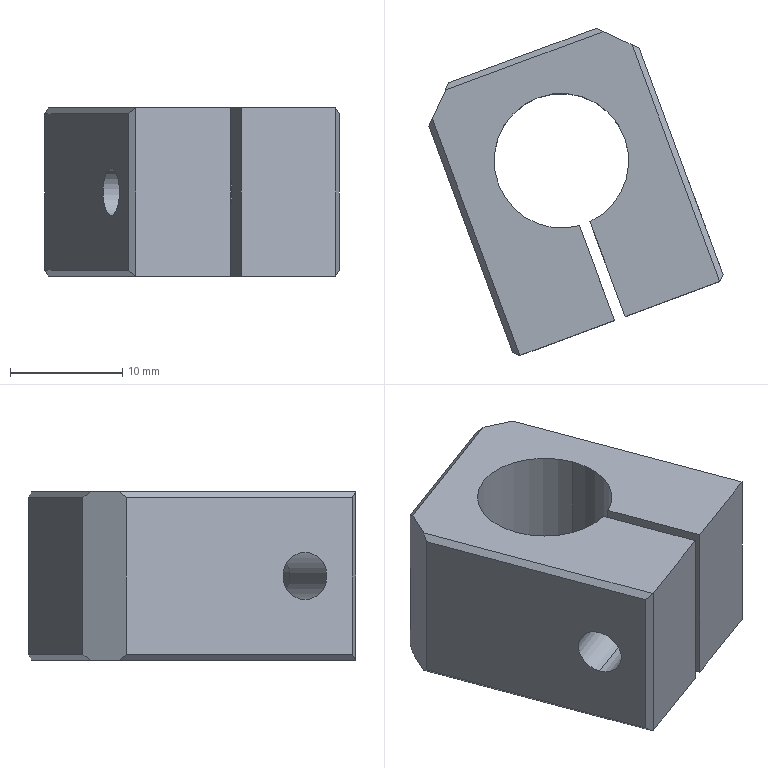Component | SolidWorks | 57-1 | 1 solid | 30 faces | box 26.22 x 29.17 x 15 mm | volume 4970 mm3 | plane 19 | cylinder 9 | cone 2 | commonest cylinder face diameters 12 x3 4.2 x2 8.7 x2 5.3 x2
build123d program:
from build123d import *

# Parameters (mm, degrees)
BOSS_EXTRUDE1_DEPTH   = 15
CHAMFER1_SIZE         = 3
M5_TAPPED_HOLE1_D     = 4.2
M5_TAPPED_HOLE1_DEPTH = 14
M5_TAPPED_HOLE1_TIP   = 1.262
CHAMFER2_SIZE         = 0.5


with BuildPart() as part:
    # Sketch1 → Boss-Extrude1 (new body)
    with BuildSketch(Plane.XY):
        with BuildLine():
            Line((0.5, -5), (10, -5))
            Line((10, -5), (10, 20))
            Line((10, 20), (-10, 20))
            Line((-10, 20), (-10, -5))
            Line((-10, -5), (-0.5, -5))
            Line((-0.5, -5), (-0.5, 4.021))
            ThreePointArc((-0.5, 4.021), (0, 16), (0.5, 4.021))
            Line((0.5, 4.021), (0.5, -5))
        make_face()
    extrude(amount=BOSS_EXTRUDE1_DEPTH)

    # Chamfer1
    chamfer1_edges = [part.edges().sort_by_distance(p)[0] for p in [
        (-10, 20, 7.5),
        (10, 20, 7.5),
    ]]
    chamfer(chamfer1_edges, length=CHAMFER1_SIZE)

    # Sketch2 → Hole1 (revolve, cut)
    with BuildSketch(Plane(origin=(10, 0, 7.5), x_dir=(0, 0, -1), z_dir=(0, 1, 0))):
        Polygon((0, 0), (0, 9.5), (2.65, 9.5), (2.65, 6.021), (4.35, 5), (4.35, 0), align=None)
    revolve(axis=Axis((16.13, 0, 7.5), (-1, 0, 0)), mode=Mode.SUBTRACT)

    # M5 Tapped Hole1
    with Locations(Plane(origin=(-0.5, 0, 0), x_dir=(0, 0, -1), z_dir=(1, 0, 0))):
        with Locations((-7.5, 0)):
            Hole(M5_TAPPED_HOLE1_D / 2, depth=M5_TAPPED_HOLE1_DEPTH)
            with Locations((0, 0, -(M5_TAPPED_HOLE1_DEPTH + M5_TAPPED_HOLE1_TIP / 2))):  # 118° drill point
                Cone(0, M5_TAPPED_HOLE1_D / 2, M5_TAPPED_HOLE1_TIP, mode=Mode.SUBTRACT)

    # Chamfer2
    chamfer2_edges = [part.edges().sort_by_distance(p)[0] for p in [
        (10, -5, 7.5),
        (-10, -5, 7.5),
        (10, 6, 15),
        (-10, 6, 0),
        (-10, 6, 15),
        (0, 20, 0),
        (0, 20, 15),
        (10, 6, 0),
    ]]
    chamfer(chamfer2_edges, length=CHAMFER2_SIZE)


solid = part.part

# Placed as in the assembly
solid = solid.moved(Location((3.473, -47.377, 51.954), (0, 0, 20.325)))
STEP:
#1=COLOUR_RGB('',0.7922,0.8196,0.9333);
#2=FILL_AREA_STYLE_COLOUR('',#1);
#3=FILL_AREA_STYLE('',(#2));
#4=SURFACE_STYLE_FILL_AREA(#3);
#5=SURFACE_SIDE_STYLE('',(#4));
#6=SURFACE_STYLE_USAGE(.BOTH.,#5);
#7=PRESENTATION_STYLE_ASSIGNMENT((#6));
#8=CARTESIAN_POINT('',(-0.2324,-2.002,2.423));
#9=VERTEX_POINT('',#8);
#10=CARTESIAN_POINT('',(-0.2324,-2.002,2.258));
#11=VERTEX_POINT('',#10);
#12=CARTESIAN_POINT('',(-0.2324,-2.002,2.341));
#13=DIRECTION('',(0.9377,0.3473,0.));
#14=DIRECTION('',(-0.3473,0.9377,0.));
#15=AXIS2_PLACEMENT_3D('',#12,#13,#14);
#16=CIRCLE('',#15,0.08268);
#17=EDGE_CURVE('',#9,#11,#16,.T.);
#18=ORIENTED_EDGE('',*,*,#17,.F.);
#19=CARTESIAN_POINT('',(0.1183,-1.872,2.423));
#20=VERTEX_POINT('',#19);
#21=CARTESIAN_POINT('',(0.1183,-1.872,2.423));
#22=DIRECTION('',(0.9377,0.3473,0.));
#23=VECTOR('',#22,39.37);
#24=LINE('',#21,#23);
#25=EDGE_CURVE('',#9,#20,#24,.T.);
#26=ORIENTED_EDGE('',*,*,#25,.T.);
#27=CARTESIAN_POINT('',(0.1183,-1.872,2.258));
#28=VERTEX_POINT('',#27);
#29=CARTESIAN_POINT('',(0.1183,-1.872,2.341));
#30=DIRECTION('',(0.9377,0.3473,0.));
#31=DIRECTION('',(0.,0.,-1.));
#32=AXIS2_PLACEMENT_3D('',#29,#30,#31);
#33=CIRCLE('',#32,0.08268);
#34=EDGE_CURVE('',#20,#28,#33,.T.);
#35=ORIENTED_EDGE('',*,*,#34,.T.);
#36=CARTESIAN_POINT('',(0.1183,-1.872,2.258));
#37=DIRECTION('',(0.9377,0.3473,0.));
#38=VECTOR('',#37,39.37);
#39=LINE('',#36,#38);
#40=EDGE_CURVE('',#11,#28,#39,.T.);
#41=ORIENTED_EDGE('',*,*,#40,.F.);
#42=EDGE_LOOP('',(#18,#26,#35,#41));
#43=FACE_OUTER_BOUND('',#42,.T.);
#44=CARTESIAN_POINT('',(0.1183,-1.872,2.341));
#45=DIRECTION('',(0.9377,0.3473,0.));
#46=DIRECTION('',(0.,0.,-1.));
#47=AXIS2_PLACEMENT_3D('',#44,#45,#46);
#48=CYLINDRICAL_SURFACE('',#47,0.08268);
#49=ADVANCED_FACE('',(#43),#48,.F.);
#50=CARTESIAN_POINT('',(0.3213,-1.797,2.512));
#51=VERTEX_POINT('',#50);
#52=CARTESIAN_POINT('',(0.3213,-1.797,2.169));
#53=VERTEX_POINT('',#52);
#54=CARTESIAN_POINT('',(0.3213,-1.797,2.341));
#55=DIRECTION('',(0.9377,0.3473,0.));
#56=DIRECTION('',(0.,0.,-1.));
#57=AXIS2_PLACEMENT_3D('',#54,#55,#56);
#58=CIRCLE('',#57,0.1713);
#59=EDGE_CURVE('',#51,#53,#58,.T.);
#60=ORIENTED_EDGE('',*,*,#59,.F.);
#61=CARTESIAN_POINT('',(0.5059,-1.728,2.512));
#62=VERTEX_POINT('',#61);
#63=CARTESIAN_POINT('',(0.5059,-1.728,2.512));
#64=DIRECTION('',(0.9377,0.3473,0.));
#65=VECTOR('',#64,39.37);
#66=LINE('',#63,#65);
#67=EDGE_CURVE('',#51,#62,#66,.T.);
#68=ORIENTED_EDGE('',*,*,#67,.T.);
#69=CARTESIAN_POINT('',(0.5059,-1.728,2.169));
#70=VERTEX_POINT('',#69);
#71=CARTESIAN_POINT('',(0.5059,-1.728,2.341));
#72=DIRECTION('',(0.9377,0.3473,0.));
#73=DIRECTION('',(0.,0.,-1.));
#74=AXIS2_PLACEMENT_3D('',#71,#72,#73);
#75=CIRCLE('',#74,0.1713);
#76=EDGE_CURVE('',#62,#70,#75,.T.);
#77=ORIENTED_EDGE('',*,*,#76,.T.);
#78=CARTESIAN_POINT('',(0.5059,-1.728,2.169));
#79=DIRECTION('',(0.9377,0.3473,0.));
#80=VECTOR('',#79,39.37);
#81=LINE('',#78,#80);
#82=EDGE_CURVE('',#53,#70,#81,.T.);
#83=ORIENTED_EDGE('',*,*,#82,.F.);
#84=EDGE_LOOP('',(#60,#68,#77,#83));
#85=FACE_OUTER_BOUND('',#84,.T.);
#86=CARTESIAN_POINT('',(0.5059,-1.728,2.341));
#87=DIRECTION('',(0.9377,0.3473,0.));
#88=DIRECTION('',(0.,0.,-1.));
#89=AXIS2_PLACEMENT_3D('',#86,#87,#88);
#90=CYLINDRICAL_SURFACE('',#89,0.1713);
#91=ADVANCED_FACE('',(#85),#90,.F.);
#92=CARTESIAN_POINT('',(0.2836,-1.811,2.445));
#93=VERTEX_POINT('',#92);
#94=CARTESIAN_POINT('',(0.2836,-1.811,2.236));
#95=VERTEX_POINT('',#94);
#96=CARTESIAN_POINT('',(0.2836,-1.811,2.341));
#97=DIRECTION('',(0.9377,0.3473,0.));
#98=DIRECTION('',(0.,0.,-1.));
#99=AXIS2_PLACEMENT_3D('',#96,#97,#98);
#100=CIRCLE('',#99,0.1043);
#101=EDGE_CURVE('',#93,#95,#100,.T.);
#102=ORIENTED_EDGE('',*,*,#101,.F.);
#103=CARTESIAN_POINT('',(0.3213,-1.797,2.512));
#104=DIRECTION('',(0.483,0.1789,0.8572));
#105=VECTOR('',#104,39.37);
#106=LINE('',#103,#105);
#107=EDGE_CURVE('',#93,#51,#106,.T.);
#108=ORIENTED_EDGE('',*,*,#107,.T.);
#109=ORIENTED_EDGE('',*,*,#59,.T.);
#110=CARTESIAN_POINT('',(0.3213,-1.797,2.169));
#111=DIRECTION('',(0.483,0.1789,-0.8572));
#112=VECTOR('',#111,39.37);
#113=LINE('',#110,#112);
#114=EDGE_CURVE('',#95,#53,#113,.T.);
#115=ORIENTED_EDGE('',*,*,#114,.F.);
#116=EDGE_LOOP('',(#102,#108,#109,#115));
#117=FACE_OUTER_BOUND('',#116,.T.);
#118=CARTESIAN_POINT('',(0.3213,-1.797,2.341));
#119=DIRECTION('',(0.9377,0.3473,0.));
#120=DIRECTION('',(0.,0.,-1.));
#121=AXIS2_PLACEMENT_3D('',#118,#119,#120);
#122=CONICAL_SURFACE('',#121,0.1713,1.03);
#123=ADVANCED_FACE('',(#117),#122,.F.);
#124=CARTESIAN_POINT('',(0.1552,-1.858,2.445));
#125=VERTEX_POINT('',#124);
#126=CARTESIAN_POINT('',(0.1552,-1.858,2.236));
#127=VERTEX_POINT('',#126);
#128=CARTESIAN_POINT('',(0.1552,-1.858,2.341));
#129=DIRECTION('',(0.9377,0.3473,0.));
#130=DIRECTION('',(-0.3473,0.9377,0.));
#131=AXIS2_PLACEMENT_3D('',#128,#129,#130);
#132=CIRCLE('',#131,0.1043);
#133=EDGE_CURVE('',#125,#127,#132,.T.);
#134=ORIENTED_EDGE('',*,*,#133,.F.);
#135=CARTESIAN_POINT('',(0.5059,-1.728,2.445));
#136=DIRECTION('',(0.9377,0.3473,0.));
#137=VECTOR('',#136,39.37);
#138=LINE('',#135,#137);
#139=EDGE_CURVE('',#125,#93,#138,.T.);
#140=ORIENTED_EDGE('',*,*,#139,.T.);
#141=ORIENTED_EDGE('',*,*,#101,.T.);
#142=CARTESIAN_POINT('',(0.5059,-1.728,2.236));
#143=DIRECTION('',(0.9377,0.3473,0.));
#144=VECTOR('',#143,39.37);
#145=LINE('',#142,#144);
#146=EDGE_CURVE('',#127,#95,#145,.T.);
#147=ORIENTED_EDGE('',*,*,#146,.F.);
#148=EDGE_LOOP('',(#134,#140,#141,#147));
#149=FACE_OUTER_BOUND('',#148,.T.);
#150=CARTESIAN_POINT('',(0.5059,-1.728,2.341));
#151=DIRECTION('',(0.9377,0.3473,0.));
#152=DIRECTION('',(0.,0.,-1.));
#153=AXIS2_PLACEMENT_3D('',#150,#151,#152);
#154=CYLINDRICAL_SURFACE('',#153,0.1043);
#155=ADVANCED_FACE('',(#149),#154,.F.);
#156=CARTESIAN_POINT('',(0.2215,-1.414,2.636));
#157=VERTEX_POINT('',#156);
#158=CARTESIAN_POINT('',(0.1002,-1.71,2.636));
#159=VERTEX_POINT('',#158);
#160=CARTESIAN_POINT('',(0.,-1.496,2.636));
#161=DIRECTION('',(0.,0.,-1.));
#162=DIRECTION('',(0.9377,0.3473,0.));
#163=AXIS2_PLACEMENT_3D('',#160,#161,#162);
#164=CIRCLE('',#163,0.2362);
#165=EDGE_CURVE('',#157,#159,#164,.T.);
#166=ORIENTED_EDGE('',*,*,#165,.F.);
#167=CARTESIAN_POINT('',(0.2215,-1.414,2.045));
#168=VERTEX_POINT('',#167);
#169=CARTESIAN_POINT('',(0.2215,-1.414,2.636));
#170=DIRECTION('',(0.,0.,-1.));
#171=VECTOR('',#170,39.37);
#172=LINE('',#169,#171);
#173=EDGE_CURVE('',#157,#168,#172,.T.);
#174=ORIENTED_EDGE('',*,*,#173,.T.);
#175=CARTESIAN_POINT('',(0.1002,-1.71,2.045));
#176=VERTEX_POINT('',#175);
#177=CARTESIAN_POINT('',(0.,-1.496,2.045));
#178=DIRECTION('',(0.,0.,-1.));
#179=DIRECTION('',(0.9377,0.3473,0.));
#180=AXIS2_PLACEMENT_3D('',#177,#178,#179);
#181=CIRCLE('',#180,0.2362);
#182=EDGE_CURVE('',#168,#176,#181,.T.);
#183=ORIENTED_EDGE('',*,*,#182,.T.);
#184=CARTESIAN_POINT('',(0.1002,-1.71,2.636));
#185=DIRECTION('',(0.,0.,-1.));
#186=VECTOR('',#185,39.37);
#187=LINE('',#184,#186);
#188=EDGE_CURVE('',#159,#176,#187,.T.);
#189=ORIENTED_EDGE('',*,*,#188,.F.);
#190=EDGE_LOOP('',(#166,#174,#183,#189));
#191=FACE_OUTER_BOUND('',#190,.T.);
#192=CARTESIAN_POINT('',(0.,-1.496,2.636));
#193=DIRECTION('',(0.,0.,-1.));
#194=DIRECTION('',(-0.9377,-0.3473,0.));
#195=AXIS2_PLACEMENT_3D('',#192,#193,#194);
#196=CYLINDRICAL_SURFACE('',#195,0.2362);
#197=ADVANCED_FACE('',(#191),#196,.F.);
#198=ORIENTED_EDGE('',*,*,#173,.F.);
#199=CARTESIAN_POINT('',(-0.2215,-1.578,2.636));
#200=VERTEX_POINT('',#199);
#201=CARTESIAN_POINT('',(0.,-1.496,2.636));
#202=DIRECTION('',(0.,0.,-1.));
#203=DIRECTION('',(0.9377,0.3473,0.));
#204=AXIS2_PLACEMENT_3D('',#201,#202,#203);
#205=CIRCLE('',#204,0.2362);
#206=EDGE_CURVE('',#200,#157,#205,.T.);
#207=ORIENTED_EDGE('',*,*,#206,.F.);
#208=CARTESIAN_POINT('',(-0.2215,-1.578,2.045));
#209=VERTEX_POINT('',#208);
#210=CARTESIAN_POINT('',(-0.2215,-1.578,2.636));
#211=DIRECTION('',(0.,0.,-1.));
#212=VECTOR('',#211,39.37);
#213=LINE('',#210,#212);
#214=EDGE_CURVE('',#200,#209,#213,.T.);
#215=ORIENTED_EDGE('',*,*,#214,.T.);
#216=CARTESIAN_POINT('',(0.,-1.496,2.045));
#217=DIRECTION('',(0.,0.,-1.));
#218=DIRECTION('',(0.9377,0.3473,0.));
#219=AXIS2_PLACEMENT_3D('',#216,#217,#218);
#220=CIRCLE('',#219,0.2362);
#221=EDGE_CURVE('',#209,#168,#220,.T.);
#222=ORIENTED_EDGE('',*,*,#221,.T.);
#223=EDGE_LOOP('',(#198,#207,#215,#222));
#224=FACE_OUTER_BOUND('',#223,.T.);
#225=CARTESIAN_POINT('',(0.,-1.496,2.636));
#226=DIRECTION('',(0.,0.,-1.));
#227=DIRECTION('',(-0.9377,-0.3473,0.));
#228=AXIS2_PLACEMENT_3D('',#225,#226,#227);
#229=CYLINDRICAL_SURFACE('',#228,0.2362);
#230=ADVANCED_FACE('',(#224),#229,.F.);
#231=CARTESIAN_POINT('',(-0.4649,-1.374,2.616));
#232=VERTEX_POINT('',#231);
#233=CARTESIAN_POINT('',(-0.4649,-1.374,2.065));
#234=VERTEX_POINT('',#233);
#235=CARTESIAN_POINT('',(-0.4649,-1.374,2.636));
#236=DIRECTION('',(0.,0.,-1.));
#237=VECTOR('',#236,39.37);
#238=LINE('',#235,#237);
#239=EDGE_CURVE('',#232,#234,#238,.T.);
#240=ORIENTED_EDGE('',*,*,#239,.T.);
#241=CARTESIAN_POINT('',(-0.1709,-2.168,2.065));
#242=VERTEX_POINT('',#241);
#243=CARTESIAN_POINT('',(-0.5059,-1.264,2.065));
#244=DIRECTION('',(0.3473,-0.9377,0.));
#245=VECTOR('',#244,39.37);
#246=LINE('',#243,#245);
#247=EDGE_CURVE('',#234,#242,#246,.T.);
#248=ORIENTED_EDGE('',*,*,#247,.T.);
#249=CARTESIAN_POINT('',(-0.1709,-2.168,2.616));
#250=VERTEX_POINT('',#249);
#251=CARTESIAN_POINT('',(-0.1709,-2.168,2.636));
#252=DIRECTION('',(0.,0.,1.));
#253=VECTOR('',#252,39.37);
#254=LINE('',#251,#253);
#255=EDGE_CURVE('',#242,#250,#254,.T.);
#256=ORIENTED_EDGE('',*,*,#255,.T.);
#257=CARTESIAN_POINT('',(-0.4649,-1.374,2.616));
#258=DIRECTION('',(-0.3473,0.9377,0.));
#259=VECTOR('',#258,39.37);
#260=LINE('',#257,#259);
#261=EDGE_CURVE('',#250,#232,#260,.T.);
#262=ORIENTED_EDGE('',*,*,#261,.T.);
#263=EDGE_LOOP('',(#240,#248,#256,#262));
#264=FACE_OUTER_BOUND('',#263,.T.);
#265=CARTESIAN_POINT('',(-0.2324,-2.002,2.341));
#266=DIRECTION('',(0.9377,0.3473,0.));
#267=DIRECTION('',(-0.3473,0.9377,0.));
#268=AXIS2_PLACEMENT_3D('',#265,#266,#267);
#269=CIRCLE('',#268,0.08268);
#270=EDGE_CURVE('',#11,#9,#269,.T.);
#271=ORIENTED_EDGE('',*,*,#270,.T.);
#272=ORIENTED_EDGE('',*,*,#17,.T.);
#273=EDGE_LOOP('',(#271,#272));
#274=FACE_BOUND('',#273,.T.);
#275=CARTESIAN_POINT('',(-0.5059,-1.264,2.636));
#276=DIRECTION('',(0.9377,0.3473,0.));
#277=DIRECTION('',(-0.3473,0.9377,0.));
#278=AXIS2_PLACEMENT_3D('',#275,#276,#277);
#279=PLANE('',#278);
#280=ADVANCED_FACE('',(#264,#274),#279,.F.);
#281=CARTESIAN_POINT('',(-0.1456,-2.18,2.636));
#282=VERTEX_POINT('',#281);
#283=CARTESIAN_POINT('',(0.1867,-2.057,2.636));
#284=VERTEX_POINT('',#283);
#285=CARTESIAN_POINT('',(-0.1641,-2.187,2.636));
#286=DIRECTION('',(0.9377,0.3473,0.));
#287=VECTOR('',#286,39.37);
#288=LINE('',#285,#287);
#289=EDGE_CURVE('',#282,#284,#288,.T.);
#290=ORIENTED_EDGE('',*,*,#289,.F.);
#291=CARTESIAN_POINT('',(-0.1456,-2.18,2.045));
#292=VERTEX_POINT('',#291);
#293=CARTESIAN_POINT('',(-0.1456,-2.18,2.636));
#294=DIRECTION('',(0.,0.,-1.));
#295=VECTOR('',#294,39.37);
#296=LINE('',#293,#295);
#297=EDGE_CURVE('',#282,#292,#296,.T.);
#298=ORIENTED_EDGE('',*,*,#297,.T.);
#299=CARTESIAN_POINT('',(0.1867,-2.057,2.045));
#300=VERTEX_POINT('',#299);
#301=CARTESIAN_POINT('',(-0.1641,-2.187,2.045));
#302=DIRECTION('',(0.9377,0.3473,0.));
#303=VECTOR('',#302,39.37);
#304=LINE('',#301,#303);
#305=EDGE_CURVE('',#292,#300,#304,.T.);
#306=ORIENTED_EDGE('',*,*,#305,.T.);
#307=CARTESIAN_POINT('',(0.1867,-2.057,2.636));
#308=DIRECTION('',(0.,0.,-1.));
#309=VECTOR('',#308,39.37);
#310=LINE('',#307,#309);
#311=EDGE_CURVE('',#284,#300,#310,.T.);
#312=ORIENTED_EDGE('',*,*,#311,.F.);
#313=EDGE_LOOP('',(#290,#298,#306,#312));
#314=FACE_OUTER_BOUND('',#313,.T.);
#315=CARTESIAN_POINT('',(-0.1641,-2.187,2.636));
#316=DIRECTION('',(-0.3473,0.9377,0.));
#317=DIRECTION('',(0.,0.,1.));
#318=AXIS2_PLACEMENT_3D('',#315,#316,#317);
#319=PLANE('',#318);
#320=ADVANCED_FACE('',(#314),#319,.F.);
#321=CARTESIAN_POINT('',(0.1183,-1.872,2.341));
#322=DIRECTION('',(0.9377,0.3473,0.));
#323=DIRECTION('',(0.,0.,-1.));
#324=AXIS2_PLACEMENT_3D('',#321,#322,#323);
#325=CIRCLE('',#324,0.08268);
#326=EDGE_CURVE('',#28,#20,#325,.T.);
#327=ORIENTED_EDGE('',*,*,#326,.F.);
#328=ORIENTED_EDGE('',*,*,#34,.F.);
#329=EDGE_LOOP('',(#327,#328));
#330=FACE_BOUND('',#329,.T.);
#331=CARTESIAN_POINT('',(0.06331,-1.724,2.045));
#332=VERTEX_POINT('',#331);
#333=CARTESIAN_POINT('',(0.06331,-1.724,2.045));
#334=DIRECTION('',(-0.3473,0.9377,0.));
#335=VECTOR('',#334,39.37);
#336=LINE('',#333,#335);
#337=EDGE_CURVE('',#300,#332,#336,.T.);
#338=ORIENTED_EDGE('',*,*,#337,.T.);
#339=CARTESIAN_POINT('',(0.06331,-1.724,2.636));
#340=VERTEX_POINT('',#339);
#341=CARTESIAN_POINT('',(0.06331,-1.724,2.636));
#342=DIRECTION('',(0.,0.,-1.));
#343=VECTOR('',#342,39.37);
#344=LINE('',#341,#343);
#345=EDGE_CURVE('',#340,#332,#344,.T.);
#346=ORIENTED_EDGE('',*,*,#345,.F.);
#347=CARTESIAN_POINT('',(0.06331,-1.724,2.636));
#348=DIRECTION('',(-0.3473,0.9377,0.));
#349=VECTOR('',#348,39.37);
#350=LINE('',#347,#349);
#351=EDGE_CURVE('',#284,#340,#350,.T.);
#352=ORIENTED_EDGE('',*,*,#351,.F.);
#353=ORIENTED_EDGE('',*,*,#311,.T.);
#354=EDGE_LOOP('',(#338,#346,#352,#353));
#355=FACE_OUTER_BOUND('',#354,.T.);
#356=CARTESIAN_POINT('',(0.06331,-1.724,2.636));
#357=DIRECTION('',(-0.9377,-0.3473,0.));
#358=DIRECTION('',(0.3473,-0.9377,0.));
#359=AXIS2_PLACEMENT_3D('',#356,#357,#358);
#360=PLANE('',#359);
#361=ADVANCED_FACE('',(#330,#355),#360,.F.);
#362=ORIENTED_EDGE('',*,*,#214,.F.);
#363=CARTESIAN_POINT('',(0.,-1.496,2.636));
#364=DIRECTION('',(0.,0.,-1.));
#365=DIRECTION('',(0.9377,0.3473,0.));
#366=AXIS2_PLACEMENT_3D('',#363,#364,#365);
#367=CIRCLE('',#366,0.2362);
#368=EDGE_CURVE('',#340,#200,#367,.T.);
#369=ORIENTED_EDGE('',*,*,#368,.F.);
#370=ORIENTED_EDGE('',*,*,#345,.T.);
#371=CARTESIAN_POINT('',(0.,-1.496,2.045));
#372=DIRECTION('',(0.,0.,-1.));
#373=DIRECTION('',(0.9377,0.3473,0.));
#374=AXIS2_PLACEMENT_3D('',#371,#372,#373);
#375=CIRCLE('',#374,0.2362);
#376=EDGE_CURVE('',#332,#209,#375,.T.);
#377=ORIENTED_EDGE('',*,*,#376,.T.);
#378=EDGE_LOOP('',(#362,#369,#370,#377));
#379=FACE_OUTER_BOUND('',#378,.T.);
#380=CARTESIAN_POINT('',(0.,-1.496,2.636));
#381=DIRECTION('',(0.,0.,-1.));
#382=DIRECTION('',(-0.9377,-0.3473,0.));
#383=AXIS2_PLACEMENT_3D('',#380,#381,#382);
#384=CYLINDRICAL_SURFACE('',#383,0.2362);
#385=ADVANCED_FACE('',(#379),#384,.F.);
#386=CARTESIAN_POINT('',(0.1552,-1.858,2.341));
#387=DIRECTION('',(0.9377,0.3473,0.));
#388=DIRECTION('',(-0.3473,0.9377,0.));
#389=AXIS2_PLACEMENT_3D('',#386,#387,#388);
#390=CIRCLE('',#389,0.1043);
#391=EDGE_CURVE('',#127,#125,#390,.T.);
#392=ORIENTED_EDGE('',*,*,#391,.T.);
#393=ORIENTED_EDGE('',*,*,#133,.T.);
#394=EDGE_LOOP('',(#392,#393));
#395=FACE_BOUND('',#394,.T.);
#396=CARTESIAN_POINT('',(0.2236,-2.043,2.045));
#397=VERTEX_POINT('',#396);
#398=CARTESIAN_POINT('',(0.1002,-1.71,2.045));
#399=DIRECTION('',(0.3473,-0.9377,0.));
#400=VECTOR('',#399,39.37);
#401=LINE('',#398,#400);
#402=EDGE_CURVE('',#176,#397,#401,.T.);
#403=ORIENTED_EDGE('',*,*,#402,.T.);
#404=CARTESIAN_POINT('',(0.2236,-2.043,2.636));
#405=VERTEX_POINT('',#404);
#406=CARTESIAN_POINT('',(0.2236,-2.043,2.636));
#407=DIRECTION('',(0.,0.,-1.));
#408=VECTOR('',#407,39.37);
#409=LINE('',#406,#408);
#410=EDGE_CURVE('',#405,#397,#409,.T.);
#411=ORIENTED_EDGE('',*,*,#410,.F.);
#412=CARTESIAN_POINT('',(0.1002,-1.71,2.636));
#413=DIRECTION('',(0.3473,-0.9377,0.));
#414=VECTOR('',#413,39.37);
#415=LINE('',#412,#414);
#416=EDGE_CURVE('',#159,#405,#415,.T.);
#417=ORIENTED_EDGE('',*,*,#416,.F.);
#418=ORIENTED_EDGE('',*,*,#188,.T.);
#419=EDGE_LOOP('',(#403,#411,#417,#418));
#420=FACE_OUTER_BOUND('',#419,.T.);
#421=CARTESIAN_POINT('',(0.1002,-1.71,2.636));
#422=DIRECTION('',(0.9377,0.3473,0.));
#423=DIRECTION('',(-0.3473,0.9377,0.));
#424=AXIS2_PLACEMENT_3D('',#421,#422,#423);
#425=PLANE('',#424);
#426=ADVANCED_FACE('',(#395,#420),#425,.F.);
#427=CARTESIAN_POINT('',(0.5559,-1.92,2.045));
#428=VERTEX_POINT('',#427);
#429=CARTESIAN_POINT('',(0.2236,-2.043,2.045));
#430=DIRECTION('',(0.9377,0.3473,0.));
#431=VECTOR('',#430,39.37);
#432=LINE('',#429,#431);
#433=EDGE_CURVE('',#397,#428,#432,.T.);
#434=ORIENTED_EDGE('',*,*,#433,.T.);
#435=CARTESIAN_POINT('',(0.5559,-1.92,2.636));
#436=VERTEX_POINT('',#435);
#437=CARTESIAN_POINT('',(0.5559,-1.92,2.636));
#438=DIRECTION('',(0.,0.,1.));
#439=VECTOR('',#438,39.37);
#440=LINE('',#437,#439);
#441=EDGE_CURVE('',#428,#436,#440,.T.);
#442=ORIENTED_EDGE('',*,*,#441,.T.);
#443=CARTESIAN_POINT('',(0.2236,-2.043,2.636));
#444=DIRECTION('',(0.9377,0.3473,0.));
#445=VECTOR('',#444,39.37);
#446=LINE('',#443,#445);
#447=EDGE_CURVE('',#405,#436,#446,.T.);
#448=ORIENTED_EDGE('',*,*,#447,.F.);
#449=ORIENTED_EDGE('',*,*,#410,.T.);
#450=EDGE_LOOP('',(#434,#442,#448,#449));
#451=FACE_OUTER_BOUND('',#450,.T.);
#452=CARTESIAN_POINT('',(0.2236,-2.043,2.636));
#453=DIRECTION('',(-0.3473,0.9377,0.));
#454=DIRECTION('',(0.,0.,1.));
#455=AXIS2_PLACEMENT_3D('',#452,#453,#454);
#456=PLANE('',#455);
#457=ADVANCED_FACE('',(#451),#456,.F.);
#458=CARTESIAN_POINT('',(0.5059,-1.728,2.341));
#459=DIRECTION('',(0.9377,0.3473,0.));
#460=DIRECTION('',(0.,0.,-1.));
#461=AXIS2_PLACEMENT_3D('',#458,#459,#460);
#462=CIRCLE('',#461,0.1713);
#463=EDGE_CURVE('',#70,#62,#462,.T.);
#464=ORIENTED_EDGE('',*,*,#463,.F.);
#465=ORIENTED_EDGE('',*,*,#76,.F.);
#466=EDGE_LOOP('',(#464,#465));
#467=FACE_BOUND('',#466,.T.);
#468=CARTESIAN_POINT('',(0.5675,-1.895,2.616));
#469=VERTEX_POINT('',#468);
#470=CARTESIAN_POINT('',(0.5675,-1.895,2.065));
#471=VERTEX_POINT('',#470);
#472=CARTESIAN_POINT('',(0.5675,-1.895,2.636));
#473=DIRECTION('',(0.,0.,-1.));
#474=VECTOR('',#473,39.37);
#475=LINE('',#472,#474);
#476=EDGE_CURVE('',#469,#471,#475,.T.);
#477=ORIENTED_EDGE('',*,*,#476,.T.);
#478=CARTESIAN_POINT('',(0.2735,-1.101,2.065));
#479=VERTEX_POINT('',#478);
#480=CARTESIAN_POINT('',(0.2324,-0.9901,2.065));
#481=DIRECTION('',(-0.3473,0.9377,0.));
#482=VECTOR('',#481,39.37);
#483=LINE('',#480,#482);
#484=EDGE_CURVE('',#471,#479,#483,.T.);
#485=ORIENTED_EDGE('',*,*,#484,.T.);
#486=CARTESIAN_POINT('',(0.2735,-1.101,2.616));
#487=VERTEX_POINT('',#486);
#488=CARTESIAN_POINT('',(0.2735,-1.101,2.636));
#489=DIRECTION('',(0.,0.,1.));
#490=VECTOR('',#489,39.37);
#491=LINE('',#488,#490);
#492=EDGE_CURVE('',#479,#487,#491,.T.);
#493=ORIENTED_EDGE('',*,*,#492,.T.);
#494=CARTESIAN_POINT('',(0.5743,-1.913,2.616));
#495=DIRECTION('',(0.3473,-0.9377,0.));
#496=VECTOR('',#495,39.37);
#497=LINE('',#494,#496);
#498=EDGE_CURVE('',#487,#469,#497,.T.);
#499=ORIENTED_EDGE('',*,*,#498,.T.);
#500=EDGE_LOOP('',(#477,#485,#493,#499));
#501=FACE_OUTER_BOUND('',#500,.T.);
#502=CARTESIAN_POINT('',(0.2324,-0.9901,2.636));
#503=DIRECTION('',(-0.9377,-0.3473,0.));
#504=DIRECTION('',(0.3473,-0.9377,0.));
#505=AXIS2_PLACEMENT_3D('',#502,#503,#504);
#506=PLANE('',#505);
#507=ADVANCED_FACE('',(#467,#501),#506,.F.);
#508=CARTESIAN_POINT('',(-0.3952,-1.223,2.065));
#509=VERTEX_POINT('',#508);
#510=CARTESIAN_POINT('',(-0.3952,-1.223,2.616));
#511=VERTEX_POINT('',#510);
#512=CARTESIAN_POINT('',(-0.3952,-1.223,2.636));
#513=DIRECTION('',(0.,0.,1.));
#514=VECTOR('',#513,39.37);
#515=LINE('',#512,#514);
#516=EDGE_CURVE('',#509,#511,#515,.T.);
#517=ORIENTED_EDGE('',*,*,#516,.T.);
#518=CARTESIAN_POINT('',(0.1217,-1.031,2.616));
#519=VERTEX_POINT('',#518);
#520=CARTESIAN_POINT('',(0.1217,-1.031,2.616));
#521=DIRECTION('',(0.9377,0.3473,0.));
#522=VECTOR('',#521,39.37);
#523=LINE('',#520,#522);
#524=EDGE_CURVE('',#511,#519,#523,.T.);
#525=ORIENTED_EDGE('',*,*,#524,.T.);
#526=CARTESIAN_POINT('',(0.1217,-1.031,2.065));
#527=VERTEX_POINT('',#526);
#528=CARTESIAN_POINT('',(0.1217,-1.031,2.636));
#529=DIRECTION('',(0.,0.,-1.));
#530=VECTOR('',#529,39.37);
#531=LINE('',#528,#530);
#532=EDGE_CURVE('',#519,#527,#531,.T.);
#533=ORIENTED_EDGE('',*,*,#532,.T.);
#534=CARTESIAN_POINT('',(-0.5059,-1.264,2.065));
#535=DIRECTION('',(-0.9377,-0.3473,0.));
#536=VECTOR('',#535,39.37);
#537=LINE('',#534,#536);
#538=EDGE_CURVE('',#527,#509,#537,.T.);
#539=ORIENTED_EDGE('',*,*,#538,.T.);
#540=EDGE_LOOP('',(#517,#525,#533,#539));
#541=FACE_OUTER_BOUND('',#540,.T.);
#542=CARTESIAN_POINT('',(-0.5059,-1.264,2.636));
#543=DIRECTION('',(0.3473,-0.9377,0.));
#544=DIRECTION('',(0.,0.,-1.));
#545=AXIS2_PLACEMENT_3D('',#542,#543,#544);
#546=PLANE('',#545);
#547=ADVANCED_FACE('',(#541),#546,.F.);
#548=CARTESIAN_POINT('',(0.2482,-1.089,2.636));
#549=VERTEX_POINT('',#548);
#550=CARTESIAN_POINT('',(0.147,-1.043,2.636));
#551=VERTEX_POINT('',#550);
#552=CARTESIAN_POINT('',(0.1976,-1.066,2.636));
#553=DIRECTION('',(-0.9087,0.4175,0.));
#554=VECTOR('',#553,39.37);
#555=LINE('',#552,#554);
#556=EDGE_CURVE('',#549,#551,#555,.T.);
#557=ORIENTED_EDGE('',*,*,#556,.T.);
#558=CARTESIAN_POINT('',(-0.4068,-1.248,2.636));
#559=VERTEX_POINT('',#558);
#560=CARTESIAN_POINT('',(-0.3883,-1.241,2.636));
#561=DIRECTION('',(-0.9377,-0.3473,0.));
#562=VECTOR('',#561,39.37);
#563=LINE('',#560,#562);
#564=EDGE_CURVE('',#551,#559,#563,.T.);
#565=ORIENTED_EDGE('',*,*,#564,.T.);
#566=CARTESIAN_POINT('',(-0.4533,-1.349,2.636));
#567=VERTEX_POINT('',#566);
#568=CARTESIAN_POINT('',(-0.43,-1.298,2.636));
#569=DIRECTION('',(-0.4175,-0.9087,0.));
#570=VECTOR('',#569,39.37);
#571=LINE('',#568,#570);
#572=EDGE_CURVE('',#559,#567,#571,.T.);
#573=ORIENTED_EDGE('',*,*,#572,.T.);
#574=CARTESIAN_POINT('',(-0.1456,-2.18,2.636));
#575=DIRECTION('',(0.3473,-0.9377,0.));
#576=VECTOR('',#575,39.37);
#577=LINE('',#574,#576);
#578=EDGE_CURVE('',#567,#282,#577,.T.);
#579=ORIENTED_EDGE('',*,*,#578,.T.);
#580=ORIENTED_EDGE('',*,*,#289,.T.);
#581=ORIENTED_EDGE('',*,*,#351,.T.);
#582=ORIENTED_EDGE('',*,*,#368,.T.);
#583=ORIENTED_EDGE('',*,*,#206,.T.);
#584=ORIENTED_EDGE('',*,*,#165,.T.);
#585=ORIENTED_EDGE('',*,*,#416,.T.);
#586=ORIENTED_EDGE('',*,*,#447,.T.);
#587=CARTESIAN_POINT('',(0.255,-1.108,2.636));
#588=DIRECTION('',(-0.3473,0.9377,0.));
#589=VECTOR('',#588,39.37);
#590=LINE('',#587,#589);
#591=EDGE_CURVE('',#436,#549,#590,.T.);
#592=ORIENTED_EDGE('',*,*,#591,.T.);
#593=EDGE_LOOP('',(#557,#565,#573,#579,#580,#581,#582,#583,#584,#585,#586,#592));
#594=FACE_OUTER_BOUND('',#593,.T.);
#595=CARTESIAN_POINT('',(0.,-1.496,2.636));
#596=DIRECTION('',(0.,0.,1.));
#597=DIRECTION('',(0.9377,0.3473,0.));
#598=AXIS2_PLACEMENT_3D('',#595,#596,#597);
#599=PLANE('',#598);
#600=ADVANCED_FACE('',(#594),#599,.T.);
#601=CARTESIAN_POINT('',(-0.4533,-1.349,2.045));
#602=VERTEX_POINT('',#601);
#603=CARTESIAN_POINT('',(-0.4068,-1.248,2.045));
#604=VERTEX_POINT('',#603);
#605=CARTESIAN_POINT('',(-0.4649,-1.374,2.045));
#606=DIRECTION('',(0.4175,0.9087,0.));
#607=VECTOR('',#606,39.37);
#608=LINE('',#605,#607);
#609=EDGE_CURVE('',#602,#604,#608,.T.);
#610=ORIENTED_EDGE('',*,*,#609,.T.);
#611=CARTESIAN_POINT('',(0.147,-1.043,2.045));
#612=VERTEX_POINT('',#611);
#613=CARTESIAN_POINT('',(-0.1299,-1.145,2.045));
#614=DIRECTION('',(0.9377,0.3473,0.));
#615=VECTOR('',#614,39.37);
#616=LINE('',#613,#615);
#617=EDGE_CURVE('',#604,#612,#616,.T.);
#618=ORIENTED_EDGE('',*,*,#617,.T.);
#619=CARTESIAN_POINT('',(0.2482,-1.089,2.045));
#620=VERTEX_POINT('',#619);
#621=CARTESIAN_POINT('',(0.1217,-1.031,2.045));
#622=DIRECTION('',(0.9087,-0.4175,0.));
#623=VECTOR('',#622,39.37);
#624=LINE('',#621,#623);
#625=EDGE_CURVE('',#612,#620,#624,.T.);
#626=ORIENTED_EDGE('',*,*,#625,.T.);
#627=CARTESIAN_POINT('',(0.3507,-1.366,2.045));
#628=DIRECTION('',(0.3473,-0.9377,0.));
#629=VECTOR('',#628,39.37);
#630=LINE('',#627,#629);
#631=EDGE_CURVE('',#620,#428,#630,.T.);
#632=ORIENTED_EDGE('',*,*,#631,.T.);
#633=ORIENTED_EDGE('',*,*,#433,.F.);
#634=ORIENTED_EDGE('',*,*,#402,.F.);
#635=ORIENTED_EDGE('',*,*,#182,.F.);
#636=ORIENTED_EDGE('',*,*,#221,.F.);
#637=ORIENTED_EDGE('',*,*,#376,.F.);
#638=ORIENTED_EDGE('',*,*,#337,.F.);
#639=ORIENTED_EDGE('',*,*,#305,.F.);
#640=CARTESIAN_POINT('',(-0.3507,-1.626,2.045));
#641=DIRECTION('',(-0.3473,0.9377,0.));
#642=VECTOR('',#641,39.37);
#643=LINE('',#640,#642);
#644=EDGE_CURVE('',#292,#602,#643,.T.);
#645=ORIENTED_EDGE('',*,*,#644,.T.);
#646=EDGE_LOOP('',(#610,#618,#626,#632,#633,#634,#635,#636,#637,#638,#639,#645));
#647=FACE_OUTER_BOUND('',#646,.T.);
#648=CARTESIAN_POINT('',(0.,-1.496,2.045));
#649=DIRECTION('',(0.,0.,1.));
#650=DIRECTION('',(0.9377,0.3473,0.));
#651=AXIS2_PLACEMENT_3D('',#648,#649,#650);
#652=PLANE('',#651);
#653=ADVANCED_FACE('',(#647),#652,.F.);
#654=ORIENTED_EDGE('',*,*,#572,.F.);
#655=CARTESIAN_POINT('',(-0.4455,-1.332,2.702));
#656=DIRECTION('',(0.3409,0.7419,-0.5774));
#657=VECTOR('',#656,39.37);
#658=LINE('',#655,#657);
#659=EDGE_CURVE('',#559,#511,#658,.T.);
#660=ORIENTED_EDGE('',*,*,#659,.T.);
#661=ORIENTED_EDGE('',*,*,#516,.F.);
#662=CARTESIAN_POINT('',(-0.3293,-1.079,2.177));
#663=DIRECTION('',(-0.3409,-0.7419,-0.5774));
#664=VECTOR('',#663,39.37);
#665=LINE('',#662,#664);
#666=EDGE_CURVE('',#509,#604,#665,.T.);
#667=ORIENTED_EDGE('',*,*,#666,.T.);
#668=ORIENTED_EDGE('',*,*,#609,.F.);
#669=CARTESIAN_POINT('',(-0.5773,-1.619,2.255));
#670=DIRECTION('',(-0.3409,-0.7419,0.5774));
#671=VECTOR('',#670,39.37);
#672=LINE('',#669,#671);
#673=EDGE_CURVE('',#602,#234,#672,.T.);
#674=ORIENTED_EDGE('',*,*,#673,.T.);
#675=ORIENTED_EDGE('',*,*,#239,.F.);
#676=CARTESIAN_POINT('',(-0.461,-1.366,2.623));
#677=DIRECTION('',(0.3409,0.7419,0.5774));
#678=VECTOR('',#677,39.37);
#679=LINE('',#676,#678);
#680=EDGE_CURVE('',#232,#567,#679,.T.);
#681=ORIENTED_EDGE('',*,*,#680,.T.);
#682=EDGE_LOOP('',(#654,#660,#661,#667,#668,#674,#675,#681));
#683=FACE_OUTER_BOUND('',#682,.T.);
#684=CARTESIAN_POINT('',(-0.4649,-1.374,2.636));
#685=DIRECTION('',(0.9087,-0.4175,0.));
#686=DIRECTION('',(0.,0.,-1.));
#687=AXIS2_PLACEMENT_3D('',#684,#685,#686);
#688=PLANE('',#687);
#689=ADVANCED_FACE('',(#683),#688,.F.);
#690=ORIENTED_EDGE('',*,*,#532,.F.);
#691=CARTESIAN_POINT('',(0.1301,-1.035,2.623));
#692=DIRECTION('',(0.7419,-0.3409,0.5774));
#693=VECTOR('',#692,39.37);
#694=LINE('',#691,#693);
#695=EDGE_CURVE('',#519,#551,#694,.T.);
#696=ORIENTED_EDGE('',*,*,#695,.T.);
#697=ORIENTED_EDGE('',*,*,#556,.F.);
#698=CARTESIAN_POINT('',(0.1638,-1.051,2.702));
#699=DIRECTION('',(0.7419,-0.3409,-0.5774));
#700=VECTOR('',#699,39.37);
#701=LINE('',#698,#700);
#702=EDGE_CURVE('',#549,#487,#701,.T.);
#703=ORIENTED_EDGE('',*,*,#702,.T.);
#704=ORIENTED_EDGE('',*,*,#492,.F.);
#705=CARTESIAN_POINT('',(0.4168,-1.167,2.177));
#706=DIRECTION('',(-0.7419,0.3409,-0.5774));
#707=VECTOR('',#706,39.37);
#708=LINE('',#705,#707);
#709=EDGE_CURVE('',#479,#620,#708,.T.);
#710=ORIENTED_EDGE('',*,*,#709,.T.);
#711=ORIENTED_EDGE('',*,*,#625,.F.);
#712=CARTESIAN_POINT('',(-0.1229,-0.9188,2.255));
#713=DIRECTION('',(-0.7419,0.3409,0.5774));
#714=VECTOR('',#713,39.37);
#715=LINE('',#712,#714);
#716=EDGE_CURVE('',#612,#527,#715,.T.);
#717=ORIENTED_EDGE('',*,*,#716,.T.);
#718=EDGE_LOOP('',(#690,#696,#697,#703,#704,#710,#711,#717));
#719=FACE_OUTER_BOUND('',#718,.T.);
#720=CARTESIAN_POINT('',(0.1217,-1.031,2.636));
#721=DIRECTION('',(-0.4175,-0.9087,0.));
#722=DIRECTION('',(0.,0.,-1.));
#723=AXIS2_PLACEMENT_3D('',#720,#721,#722);
#724=PLANE('',#723);
#725=ADVANCED_FACE('',(#719),#724,.F.);
#726=ORIENTED_EDGE('',*,*,#139,.F.);
#727=ORIENTED_EDGE('',*,*,#391,.F.);
#728=ORIENTED_EDGE('',*,*,#146,.T.);
#729=CARTESIAN_POINT('',(0.2836,-1.811,2.341));
#730=DIRECTION('',(0.9377,0.3473,0.));
#731=DIRECTION('',(0.,0.,-1.));
#732=AXIS2_PLACEMENT_3D('',#729,#730,#731);
#733=CIRCLE('',#732,0.1043);
#734=EDGE_CURVE('',#95,#93,#733,.T.);
#735=ORIENTED_EDGE('',*,*,#734,.T.);
#736=EDGE_LOOP('',(#726,#727,#728,#735));
#737=FACE_OUTER_BOUND('',#736,.T.);
#738=CARTESIAN_POINT('',(0.5059,-1.728,2.341));
#739=DIRECTION('',(0.9377,0.3473,0.));
#740=DIRECTION('',(0.,0.,-1.));
#741=AXIS2_PLACEMENT_3D('',#738,#739,#740);
#742=CYLINDRICAL_SURFACE('',#741,0.1043);
#743=ADVANCED_FACE('',(#737),#742,.F.);
#744=ORIENTED_EDGE('',*,*,#107,.F.);
#745=ORIENTED_EDGE('',*,*,#734,.F.);
#746=ORIENTED_EDGE('',*,*,#114,.T.);
#747=CARTESIAN_POINT('',(0.3213,-1.797,2.341));
#748=DIRECTION('',(0.9377,0.3473,0.));
#749=DIRECTION('',(0.,0.,-1.));
#750=AXIS2_PLACEMENT_3D('',#747,#748,#749);
#751=CIRCLE('',#750,0.1713);
#752=EDGE_CURVE('',#53,#51,#751,.T.);
#753=ORIENTED_EDGE('',*,*,#752,.T.);
#754=EDGE_LOOP('',(#744,#745,#746,#753));
#755=FACE_OUTER_BOUND('',#754,.T.);
#756=CARTESIAN_POINT('',(0.3213,-1.797,2.341));
#757=DIRECTION('',(0.9377,0.3473,0.));
#758=DIRECTION('',(0.,0.,-1.));
#759=AXIS2_PLACEMENT_3D('',#756,#757,#758);
#760=CONICAL_SURFACE('',#759,0.1713,1.03);
#761=ADVANCED_FACE('',(#755),#760,.F.);
#762=ORIENTED_EDGE('',*,*,#67,.F.);
#763=ORIENTED_EDGE('',*,*,#752,.F.);
#764=ORIENTED_EDGE('',*,*,#82,.T.);
#765=ORIENTED_EDGE('',*,*,#463,.T.);
#766=EDGE_LOOP('',(#762,#763,#764,#765));
#767=FACE_OUTER_BOUND('',#766,.T.);
#768=CARTESIAN_POINT('',(0.5059,-1.728,2.341));
#769=DIRECTION('',(0.9377,0.3473,0.));
#770=DIRECTION('',(0.,0.,-1.));
#771=AXIS2_PLACEMENT_3D('',#768,#769,#770);
#772=CYLINDRICAL_SURFACE('',#771,0.1713);
#773=ADVANCED_FACE('',(#767),#772,.F.);
#774=ORIENTED_EDGE('',*,*,#25,.F.);
#775=ORIENTED_EDGE('',*,*,#270,.F.);
#776=ORIENTED_EDGE('',*,*,#40,.T.);
#777=ORIENTED_EDGE('',*,*,#326,.T.);
#778=EDGE_LOOP('',(#774,#775,#776,#777));
#779=FACE_OUTER_BOUND('',#778,.T.);
#780=CARTESIAN_POINT('',(0.1183,-1.872,2.341));
#781=DIRECTION('',(0.9377,0.3473,0.));
#782=DIRECTION('',(0.,0.,-1.));
#783=AXIS2_PLACEMENT_3D('',#780,#781,#782);
#784=CYLINDRICAL_SURFACE('',#783,0.08268);
#785=ADVANCED_FACE('',(#779),#784,.F.);
#786=ORIENTED_EDGE('',*,*,#695,.F.);
#787=ORIENTED_EDGE('',*,*,#524,.F.);
#788=ORIENTED_EDGE('',*,*,#659,.F.);
#789=ORIENTED_EDGE('',*,*,#564,.F.);
#790=EDGE_LOOP('',(#786,#787,#788,#789));
#791=FACE_OUTER_BOUND('',#790,.T.);
#792=CARTESIAN_POINT('',(-0.1299,-1.145,2.636));
#793=DIRECTION('',(-0.2456,0.6631,0.7071));
#794=DIRECTION('',(0.9377,0.3473,0.));
#795=AXIS2_PLACEMENT_3D('',#792,#793,#794);
#796=PLANE('',#795);
#797=ADVANCED_FACE('',(#791),#796,.T.);
#798=ORIENTED_EDGE('',*,*,#716,.F.);
#799=ORIENTED_EDGE('',*,*,#617,.F.);
#800=ORIENTED_EDGE('',*,*,#666,.F.);
#801=ORIENTED_EDGE('',*,*,#538,.F.);
#802=EDGE_LOOP('',(#798,#799,#800,#801));
#803=FACE_OUTER_BOUND('',#802,.T.);
#804=CARTESIAN_POINT('',(-0.5059,-1.264,2.065));
#805=DIRECTION('',(0.2456,-0.6631,0.7071));
#806=DIRECTION('',(-0.9377,-0.3473,0.));
#807=AXIS2_PLACEMENT_3D('',#804,#805,#806);
#808=PLANE('',#807);
#809=ADVANCED_FACE('',(#803),#808,.F.);
#810=ORIENTED_EDGE('',*,*,#680,.F.);
#811=ORIENTED_EDGE('',*,*,#261,.F.);
#812=CARTESIAN_POINT('',(-0.1456,-2.18,2.636));
#813=DIRECTION('',(-0.7419,0.3409,-0.5774));
#814=VECTOR('',#813,39.37);
#815=LINE('',#812,#814);
#816=EDGE_CURVE('',#282,#250,#815,.T.);
#817=ORIENTED_EDGE('',*,*,#816,.F.);
#818=ORIENTED_EDGE('',*,*,#578,.F.);
#819=EDGE_LOOP('',(#810,#811,#817,#818));
#820=FACE_OUTER_BOUND('',#819,.T.);
#821=CARTESIAN_POINT('',(-0.3507,-1.626,2.636));
#822=DIRECTION('',(-0.6631,-0.2456,0.7071));
#823=DIRECTION('',(-0.3473,0.9377,0.));
#824=AXIS2_PLACEMENT_3D('',#821,#822,#823);
#825=PLANE('',#824);
#826=ADVANCED_FACE('',(#820),#825,.T.);
#827=ORIENTED_EDGE('',*,*,#816,.T.);
#828=ORIENTED_EDGE('',*,*,#255,.F.);
#829=CARTESIAN_POINT('',(-0.3986,-2.064,2.242));
#830=DIRECTION('',(-0.7419,0.3409,0.5774));
#831=VECTOR('',#830,39.37);
#832=LINE('',#829,#831);
#833=EDGE_CURVE('',#292,#242,#832,.T.);
#834=ORIENTED_EDGE('',*,*,#833,.F.);
#835=ORIENTED_EDGE('',*,*,#297,.F.);
#836=EDGE_LOOP('',(#827,#828,#834,#835));
#837=FACE_OUTER_BOUND('',#836,.T.);
#838=CARTESIAN_POINT('',(-0.1456,-2.18,2.636));
#839=DIRECTION('',(0.4175,0.9087,0.));
#840=DIRECTION('',(0.,0.,-1.));
#841=AXIS2_PLACEMENT_3D('',#838,#839,#840);
#842=PLANE('',#841);
#843=ADVANCED_FACE('',(#837),#842,.F.);
#844=ORIENTED_EDGE('',*,*,#673,.F.);
#845=ORIENTED_EDGE('',*,*,#644,.F.);
#846=ORIENTED_EDGE('',*,*,#833,.T.);
#847=ORIENTED_EDGE('',*,*,#247,.F.);
#848=EDGE_LOOP('',(#844,#845,#846,#847));
#849=FACE_OUTER_BOUND('',#848,.T.);
#850=CARTESIAN_POINT('',(-0.5059,-1.264,2.065));
#851=DIRECTION('',(0.6631,0.2456,0.7071));
#852=DIRECTION('',(0.3473,-0.9377,0.));
#853=AXIS2_PLACEMENT_3D('',#850,#851,#852);
#854=PLANE('',#853);
#855=ADVANCED_FACE('',(#849),#854,.F.);
#856=ORIENTED_EDGE('',*,*,#702,.F.);
#857=ORIENTED_EDGE('',*,*,#591,.F.);
#858=CARTESIAN_POINT('',(0.6721,-1.667,2.439));
#859=DIRECTION('',(-0.3409,-0.7419,0.5774));
#860=VECTOR('',#859,39.37);
#861=LINE('',#858,#860);
#862=EDGE_CURVE('',#469,#436,#861,.T.);
#863=ORIENTED_EDGE('',*,*,#862,.F.);
#864=ORIENTED_EDGE('',*,*,#498,.F.);
#865=EDGE_LOOP('',(#856,#857,#863,#864));
#866=FACE_OUTER_BOUND('',#865,.T.);
#867=CARTESIAN_POINT('',(0.3507,-1.366,2.636));
#868=DIRECTION('',(0.6631,0.2456,0.7071));
#869=DIRECTION('',(0.3473,-0.9377,0.));
#870=AXIS2_PLACEMENT_3D('',#867,#868,#869);
#871=PLANE('',#870);
#872=ADVANCED_FACE('',(#866),#871,.T.);
#873=ORIENTED_EDGE('',*,*,#862,.T.);
#874=ORIENTED_EDGE('',*,*,#441,.F.);
#875=CARTESIAN_POINT('',(0.6798,-1.65,2.255));
#876=DIRECTION('',(-0.3409,-0.7419,-0.5774));
#877=VECTOR('',#876,39.37);
#878=LINE('',#875,#877);
#879=EDGE_CURVE('',#471,#428,#878,.T.);
#880=ORIENTED_EDGE('',*,*,#879,.F.);
#881=ORIENTED_EDGE('',*,*,#476,.F.);
#882=EDGE_LOOP('',(#873,#874,#880,#881));
#883=FACE_OUTER_BOUND('',#882,.T.);
#884=CARTESIAN_POINT('',(0.5675,-1.895,2.636));
#885=DIRECTION('',(-0.9087,0.4175,0.));
#886=DIRECTION('',(0.,0.,-1.));
#887=AXIS2_PLACEMENT_3D('',#884,#885,#886);
#888=PLANE('',#887);
#889=ADVANCED_FACE('',(#883),#888,.F.);
#890=ORIENTED_EDGE('',*,*,#879,.T.);
#891=ORIENTED_EDGE('',*,*,#631,.F.);
#892=ORIENTED_EDGE('',*,*,#709,.F.);
#893=ORIENTED_EDGE('',*,*,#484,.F.);
#894=EDGE_LOOP('',(#890,#891,#892,#893));
#895=FACE_OUTER_BOUND('',#894,.T.);
#896=CARTESIAN_POINT('',(0.2324,-0.9901,2.065));
#897=DIRECTION('',(-0.6631,-0.2456,0.7071));
#898=DIRECTION('',(-0.3473,0.9377,0.));
#899=AXIS2_PLACEMENT_3D('',#896,#897,#898);
#900=PLANE('',#899);
#901=ADVANCED_FACE('',(#895),#900,.F.);
#902=CLOSED_SHELL('',(#49,#91,#123,#155,#197,#230,#280,#320,#361,#385,#426,#457,#507,#547,#600,#653,#689,#725,#743,#761,#773,#785,#797,#809,#826,#843,#855,#872,#889,#901));
#903=MANIFOLD_SOLID_BREP('',#902);
#904=STYLED_ITEM('',(#7),#903);
#905=(LENGTH_UNIT()NAMED_UNIT(*)SI_UNIT($,.METRE.));
#906=LENGTH_MEASURE_WITH_UNIT(LENGTH_MEASURE(0.0254),#905);
#907=DIMENSIONAL_EXPONENTS(1.,0.,0.,0.,0.,0.,0.);
#908=(CONVERSION_BASED_UNIT('',#906)LENGTH_UNIT()NAMED_UNIT(#907));
#909=UNCERTAINTY_MEASURE_WITH_UNIT(LENGTH_MEASURE(0.00001),#908,'','');
#910=(NAMED_UNIT(*)PLANE_ANGLE_UNIT()SI_UNIT($,.RADIAN.));
#911=(NAMED_UNIT(*)SI_UNIT($,.STERADIAN.)SOLID_ANGLE_UNIT());
#912=(GEOMETRIC_REPRESENTATION_CONTEXT(3)GLOBAL_UNCERTAINTY_ASSIGNED_CONTEXT((#909))GLOBAL_UNIT_ASSIGNED_CONTEXT((#908,#910,#911))REPRESENTATION_CONTEXT('',''));
#913=MECHANICAL_DESIGN_GEOMETRIC_PRESENTATION_REPRESENTATION('',(#904),#912);
#914=CARTESIAN_POINT('',(0.,0.,0.));
#915=DIRECTION('',(0.,0.,1.));
#916=DIRECTION('',(1.,0.,0.));
#917=AXIS2_PLACEMENT_3D('',#914,#915,#916);
#918=(LENGTH_UNIT()NAMED_UNIT(*)SI_UNIT($,.METRE.));
#919=LENGTH_MEASURE_WITH_UNIT(LENGTH_MEASURE(0.0254),#918);
#920=DIMENSIONAL_EXPONENTS(1.,0.,0.,0.,0.,0.,0.);
#921=(CONVERSION_BASED_UNIT('',#919)LENGTH_UNIT()NAMED_UNIT(#920));
#922=UNCERTAINTY_MEASURE_WITH_UNIT(LENGTH_MEASURE(0.00001),#921,'','');
#923=(NAMED_UNIT(*)PLANE_ANGLE_UNIT()SI_UNIT($,.RADIAN.));
#924=(NAMED_UNIT(*)SI_UNIT($,.STERADIAN.)SOLID_ANGLE_UNIT());
#925=(GEOMETRIC_REPRESENTATION_CONTEXT(3)GLOBAL_UNCERTAINTY_ASSIGNED_CONTEXT((#922))GLOBAL_UNIT_ASSIGNED_CONTEXT((#921,#923,#924))REPRESENTATION_CONTEXT('',''));
#926=ADVANCED_BREP_SHAPE_REPRESENTATION('',(#903,#917),#925);
#927=PRESENTATION_LAYER_ASSIGNMENT('','',(#904));